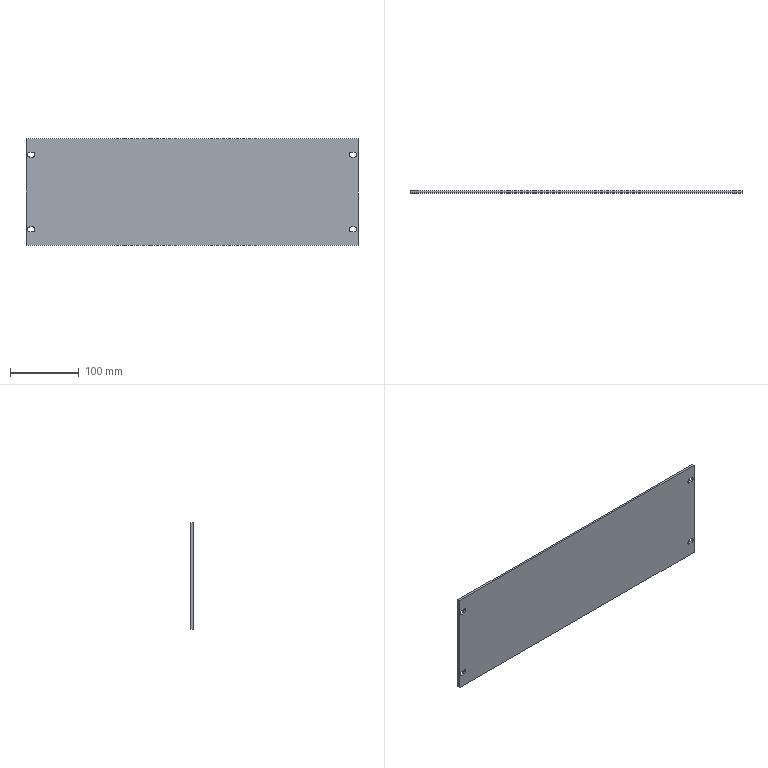Component | SolidWorks | AX00-100.1.1-1_20.1.1-1 | 1 solid | 26 faces | box 482 x 3 x 155 mm | volume 223332 mm3 | plane 14 | cylinder 12 | commonest cylinder face diameters 7 x12
build123d program:
from build123d import *

# Parameters (mm, degrees)
SKETCH1_W            = 482
SKETCH1_H            = 155
BOSS_EXTRUDE1_DEPTH  = 3
CUT_EXTRUDE1_DEPTH   = 10
MIRROR2_COPY_1_DEPTH = 10


with BuildPart() as part:
    # Sketch1 → Boss-Extrude1 (new body)
    with BuildSketch(Plane.XY):
        Rectangle(SKETCH1_W, SKETCH1_H)
    extrude(amount=BOSS_EXTRUDE1_DEPTH)

    # Sketch2 → Cut-Extrude1 (cut)
    with BuildSketch(Plane.XY.offset(3)):
        with BuildLine():
            Line((-235.5, 57.725), (-231.5, 57.725))
            ThreePointArc((-231.5, 57.725), (-228, 54.225), (-231.5, 50.725))
            Line((-231.5, 50.725), (-235.5, 50.725))
            ThreePointArc((-235.5, 50.725), (-239, 54.225), (-235.5, 57.725))
        make_face()
    cut_extrude1 = extrude(amount=-CUT_EXTRUDE1_DEPTH, mode=Mode.SUBTRACT)

    # Mirror1: Cut-Extrude1 across plane
    add(cut_extrude1.mirror(Plane.ZX), mode=Mode.SUBTRACT)

    # Mirror2: Cut-Extrude1 across plane
    add(cut_extrude1.mirror(Plane(origin=(0, 0, 0), x_dir=(0, 0, 1), z_dir=(1, 0, 0))), mode=Mode.SUBTRACT)

    # Mirror2 copy 1 sketch → Mirror2 copy 1 (cut)
    with BuildSketch(Plane(origin=(0, 0, 3), x_dir=(-1, 0, 0), z_dir=(0, 0, 1))):
        with BuildLine():
            Line((-235.5, 57.725), (-231.5, 57.725))
            ThreePointArc((-231.5, 57.725), (-228, 54.225), (-231.5, 50.725))
            Line((-231.5, 50.725), (-235.5, 50.725))
            ThreePointArc((-235.5, 50.725), (-239, 54.225), (-235.5, 57.725))
        make_face()
    extrude(amount=-MIRROR2_COPY_1_DEPTH, mode=Mode.SUBTRACT)


solid = part.part

# Placed as in the assembly
solid = solid.moved(Location((876.131, -383.636, -94), (90, 0, 0)))